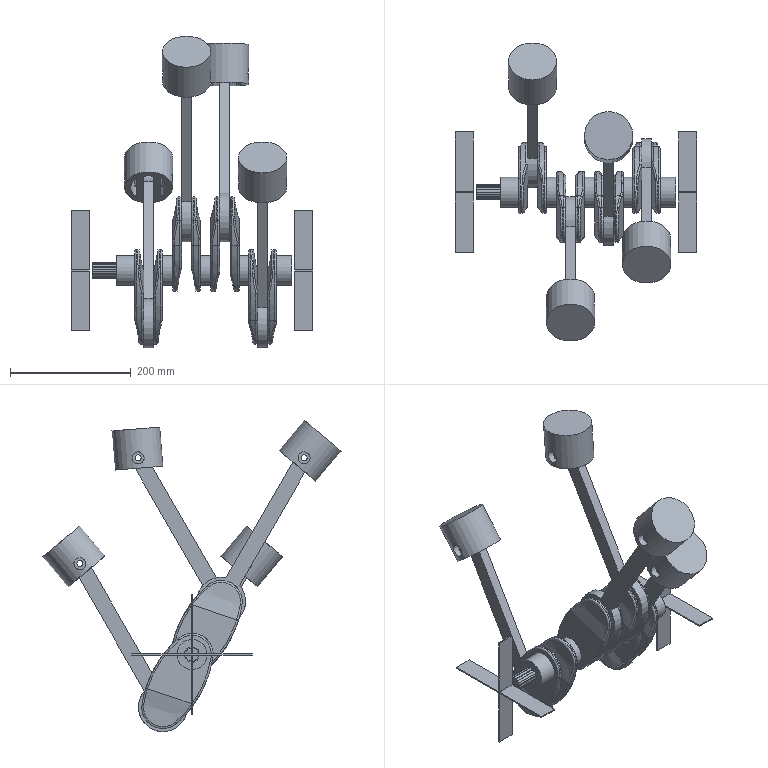Assembly | NX | mm | 15 component files | 33 solids | 440 faces | box 400 x 494.47 x 516.33 mm | volume 3190340 mm3 | plane 165 | cylinder 121 | spline 94 | torus 42 | other 18 | commonest cylinder face diameters 20 x24 362.38 x16 60 x16 70 x10 50 x9 25.4 x9 22 x9 24 x8
Bill of materials:
unnamed part 1 | 2 |  | Two separate, very thin, flat rectangular strips set apart from each other. Each strip is long and narrow, and an edge line across its width splits it into two rectangular sections.
unnamed part 2 | 4 |  | Flat link of even thickness: a straight, narrow bar with a small round eye at one end and a larger ring at the other. Both ends have through holes.
unnamed part 3 | 4 |  | Hollow cylindrical sleeve shaped like a spool, with a raised flange of the same size at each end and a straight hole running through its axis.
unnamed part 4 | 1 |  | Crankshaft-like shaft. Several journals sit on one shared axis. Four offset pins are each held between a pair of flat webs. A smaller-diameter stub sticks out from one end.
unnamed part 5 | 4 |  | Solid short cylinder with flat end faces. A small round hole runs across it, through the curved side wall, closer to one end than the other.
Mates:
1. fix | datum 2 component
2. center | datum 1 face | datum 1 face | datum 2 face | datum 2 face
3. touch align | datum 1 face | datum 2 face
4. center | datum 1 face | datum 1 face | crankshaft 1 face
5. center | crankshaft 1 face | crankshaft 1 face | datum 1 face | datum 1 face
6. center | datum 1 face | datum 1 face | crankshaft 1 face
7. center | datum 1 face | datum 1 face | datum 2 face | datum 2 face
8. concentric | con_rod 4 edge | crankshaft 1 edge
9. angle | con_rod 4 face | datum 1 face
10. touch align | piston 4 face | con_rod 4 face
11. center | con_rod 4 face | con_rod 4 face | piston 4 face | piston 4 face
12. concentric | con_rod 3 arc | crankshaft 1 edge
13. angle | con_rod 3 face | datum 1 face
14. concentric | con_rod 3 arc | piston 3 edge
15. concentric | con_rod 2 arc | crankshaft 1 edge
16. angle | datum 1 face | con_rod 2 face
17. concentric | con_rod 2 arc | piston 2 edge
18. concentric | con_rod 1 arc | crankshaft 1 edge
19. angle | con_rod 1 face | datum 1 face
20. concentric | con_rod 1 arc | piston 1 edge
21. touch align | journal 4 face | piston 4 face
22. center | journal 4 face | journal 4 face | piston 4 face
23. touch align | journal 3 face | piston 2 face
24. center | journal 3 face | journal 3 face | piston 2 face
25. center | journal 2 face | journal 2 face | piston 3 face
26. touch align | piston 3 face | journal 2 face
27. touch align | journal 1 face | piston 1 face
28. center | journal 1 face | journal 1 face | piston 1 face